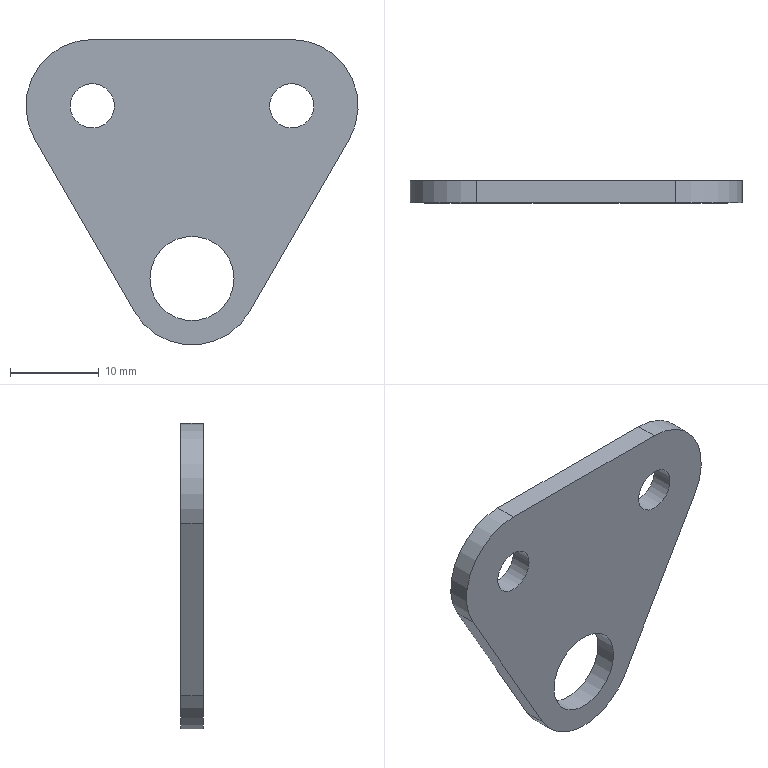Component | NX | 7 | 1 solid | 11 faces | box 37.5 x 2.5 x 34.49 mm | volume 1980 mm3 | cylinder 6 | plane 5 | commonest cylinder face diameters 15 x3 5 x2 9.5 x1
STEP:
#1=CARTESIAN_POINT('',(0.,0.,0.));
#2=DIRECTION('',(0.,0.,1.));
#3=DIRECTION('',(1.,0.,0.));
#4=AXIS2_PLACEMENT_3D('',#1,#2,#3);
#5=CARTESIAN_POINT('',(-395.181,171.749,-74.831));
#6=VERTEX_POINT('',#5);
#7=CARTESIAN_POINT('',(-388.686,171.749,-63.581));
#8=VERTEX_POINT('',#7);
#9=CARTESIAN_POINT('',(-388.686,171.749,-71.081));
#10=DIRECTION('',(0.,1.,0.));
#11=DIRECTION('',(-1.,0.,0.));
#12=AXIS2_PLACEMENT_3D('',#9,#10,#11);
#13=CIRCLE('',#12,7.5);
#14=CARTESIAN_POINT('',(-388.686,174.249,-71.081));
#15=DIRECTION('',(0.,-1.,0.));
#16=DIRECTION('',(-1.,0.,0.));
#17=AXIS2_PLACEMENT_3D('',#14,#15,#16);
#18=CYLINDRICAL_SURFACE('',#17,7.5);
#19=CARTESIAN_POINT('',(12.566,2.5));
#20=DIRECTION('',(-1.,0.));
#21=VECTOR('',#20,1.);
#22=LINE('',#19,#21);
#23=(GEOMETRIC_REPRESENTATION_CONTEXT(2)PARAMETRIC_REPRESENTATION_CONTEXT()REPRESENTATION_CONTEXT('',''));
#24=DEFINITIONAL_REPRESENTATION('',(#22),#23);
#25=PCURVE('',#18,#24);
#26=CARTESIAN_POINT('',(-388.686,171.749,-71.081));
#27=DIRECTION('',(0.,1.,0.));
#28=DIRECTION('',(1.,0.,0.));
#29=AXIS2_PLACEMENT_3D('',#26,#27,#28);
#30=PLANE('',#29);
#31=CARTESIAN_POINT('',(0.,0.));
#32=DIRECTION('',(-1.,0.));
#33=AXIS2_PLACEMENT_2D('',#31,#32);
#34=CIRCLE('',#33,7.5);
#35=(GEOMETRIC_REPRESENTATION_CONTEXT(2)PARAMETRIC_REPRESENTATION_CONTEXT()REPRESENTATION_CONTEXT('',''));
#36=DEFINITIONAL_REPRESENTATION('',(#34),#35);
#37=PCURVE('',#30,#36);
#38=SURFACE_CURVE('',#13,(#25,#37),.PCURVE_S1.);
#39=EDGE_CURVE('',#6,#8,#38,.T.);
#40=ORIENTED_EDGE('',*,*,#39,.T.);
#41=CARTESIAN_POINT('',(-388.686,174.249,-63.581));
#42=VERTEX_POINT('',#41);
#43=CARTESIAN_POINT('',(-388.686,174.249,-63.581));
#44=DIRECTION('',(0.,-1.,0.));
#45=VECTOR('',#44,1.);
#46=LINE('',#43,#45);
#47=CARTESIAN_POINT('',(4.712,0.));
#48=DIRECTION('',(0.,1.));
#49=VECTOR('',#48,1.);
#50=LINE('',#47,#49);
#51=(GEOMETRIC_REPRESENTATION_CONTEXT(2)PARAMETRIC_REPRESENTATION_CONTEXT()REPRESENTATION_CONTEXT('',''));
#52=DEFINITIONAL_REPRESENTATION('',(#50),#51);
#53=PCURVE('',#18,#52);
#54=CARTESIAN_POINT('',(-388.686,174.249,-63.581));
#55=DIRECTION('',(0.,0.,-1.));
#56=DIRECTION('',(0.,1.,0.));
#57=AXIS2_PLACEMENT_3D('',#54,#55,#56);
#58=PLANE('',#57);
#59=CARTESIAN_POINT('',(0.,0.));
#60=DIRECTION('',(-1.,0.));
#61=VECTOR('',#60,1.);
#62=LINE('',#59,#61);
#63=(GEOMETRIC_REPRESENTATION_CONTEXT(2)PARAMETRIC_REPRESENTATION_CONTEXT()REPRESENTATION_CONTEXT('',''));
#64=DEFINITIONAL_REPRESENTATION('',(#62),#63);
#65=PCURVE('',#58,#64);
#66=SURFACE_CURVE('',#46,(#53,#65),.PCURVE_S1.);
#67=EDGE_CURVE('',#42,#8,#66,.T.);
#68=ORIENTED_EDGE('',*,*,#67,.F.);
#69=CARTESIAN_POINT('',(-395.181,174.249,-74.831));
#70=VERTEX_POINT('',#69);
#71=CARTESIAN_POINT('',(-388.686,174.249,-71.081));
#72=DIRECTION('',(0.,1.,0.));
#73=DIRECTION('',(-1.,0.,0.));
#74=AXIS2_PLACEMENT_3D('',#71,#72,#73);
#75=CIRCLE('',#74,7.5);
#76=CARTESIAN_POINT('',(12.566,0.));
#77=DIRECTION('',(-1.,0.));
#78=VECTOR('',#77,1.);
#79=LINE('',#76,#78);
#80=(GEOMETRIC_REPRESENTATION_CONTEXT(2)PARAMETRIC_REPRESENTATION_CONTEXT()REPRESENTATION_CONTEXT('',''));
#81=DEFINITIONAL_REPRESENTATION('',(#79),#80);
#82=PCURVE('',#18,#81);
#83=CARTESIAN_POINT('',(-388.686,174.249,-71.081));
#84=DIRECTION('',(0.,1.,0.));
#85=DIRECTION('',(1.,0.,0.));
#86=AXIS2_PLACEMENT_3D('',#83,#84,#85);
#87=PLANE('',#86);
#88=CARTESIAN_POINT('',(0.,0.));
#89=DIRECTION('',(-1.,0.));
#90=AXIS2_PLACEMENT_2D('',#88,#89);
#91=CIRCLE('',#90,7.5);
#92=(GEOMETRIC_REPRESENTATION_CONTEXT(2)PARAMETRIC_REPRESENTATION_CONTEXT()REPRESENTATION_CONTEXT('',''));
#93=DEFINITIONAL_REPRESENTATION('',(#91),#92);
#94=PCURVE('',#87,#93);
#95=SURFACE_CURVE('',#75,(#82,#94),.PCURVE_S1.);
#96=EDGE_CURVE('',#70,#42,#95,.T.);
#97=ORIENTED_EDGE('',*,*,#96,.F.);
#98=CARTESIAN_POINT('',(-395.181,174.249,-74.831));
#99=DIRECTION('',(0.,-1.,0.));
#100=VECTOR('',#99,1.);
#101=LINE('',#98,#100);
#102=CARTESIAN_POINT('',(6.807,0.));
#103=DIRECTION('',(0.,1.));
#104=VECTOR('',#103,1.);
#105=LINE('',#102,#104);
#106=(GEOMETRIC_REPRESENTATION_CONTEXT(2)PARAMETRIC_REPRESENTATION_CONTEXT()REPRESENTATION_CONTEXT('',''));
#107=DEFINITIONAL_REPRESENTATION('',(#105),#106);
#108=PCURVE('',#18,#107);
#109=CARTESIAN_POINT('',(-383.931,174.249,-94.316));
#110=DIRECTION('',(0.866,0.,0.5));
#111=DIRECTION('',(0.5,0.,-0.866));
#112=AXIS2_PLACEMENT_3D('',#109,#110,#111);
#113=PLANE('',#112);
#114=CARTESIAN_POINT('',(-22.5,0.));
#115=DIRECTION('',(0.,-1.));
#116=VECTOR('',#115,1.);
#117=LINE('',#114,#116);
#118=(GEOMETRIC_REPRESENTATION_CONTEXT(2)PARAMETRIC_REPRESENTATION_CONTEXT()REPRESENTATION_CONTEXT('',''));
#119=DEFINITIONAL_REPRESENTATION('',(#117),#118);
#120=PCURVE('',#113,#119);
#121=SURFACE_CURVE('',#101,(#108,#120),.PCURVE_S1.);
#122=EDGE_CURVE('',#70,#6,#121,.T.);
#123=ORIENTED_EDGE('',*,*,#122,.T.);
#124=EDGE_LOOP('',(#40,#68,#97,#123));
#125=FACE_BOUND('',#124,.T.);
#126=ADVANCED_FACE('',(#125),#18,.T.);
#127=CARTESIAN_POINT('',(-366.186,171.749,-63.581));
#128=VERTEX_POINT('',#127);
#129=CARTESIAN_POINT('',(-388.686,171.749,-63.581));
#130=DIRECTION('',(1.,0.,0.));
#131=VECTOR('',#130,1.);
#132=LINE('',#129,#131);
#133=CARTESIAN_POINT('',(-2.5,0.));
#134=DIRECTION('',(0.,1.));
#135=VECTOR('',#134,1.);
#136=LINE('',#133,#135);
#137=(GEOMETRIC_REPRESENTATION_CONTEXT(2)PARAMETRIC_REPRESENTATION_CONTEXT()REPRESENTATION_CONTEXT('',''));
#138=DEFINITIONAL_REPRESENTATION('',(#136),#137);
#139=PCURVE('',#58,#138);
#140=CARTESIAN_POINT('',(0.,-7.5));
#141=DIRECTION('',(1.,0.));
#142=VECTOR('',#141,1.);
#143=LINE('',#140,#142);
#144=(GEOMETRIC_REPRESENTATION_CONTEXT(2)PARAMETRIC_REPRESENTATION_CONTEXT()REPRESENTATION_CONTEXT('',''));
#145=DEFINITIONAL_REPRESENTATION('',(#143),#144);
#146=PCURVE('',#30,#145);
#147=SURFACE_CURVE('',#132,(#139,#146),.PCURVE_S1.);
#148=EDGE_CURVE('',#8,#128,#147,.T.);
#149=ORIENTED_EDGE('',*,*,#148,.T.);
#150=CARTESIAN_POINT('',(-366.186,174.249,-63.581));
#151=VERTEX_POINT('',#150);
#152=CARTESIAN_POINT('',(-366.186,174.249,-63.581));
#153=DIRECTION('',(0.,-1.,0.));
#154=VECTOR('',#153,1.);
#155=LINE('',#152,#154);
#156=CARTESIAN_POINT('',(0.,22.5));
#157=DIRECTION('',(-1.,0.));
#158=VECTOR('',#157,1.);
#159=LINE('',#156,#158);
#160=(GEOMETRIC_REPRESENTATION_CONTEXT(2)PARAMETRIC_REPRESENTATION_CONTEXT()REPRESENTATION_CONTEXT('',''));
#161=DEFINITIONAL_REPRESENTATION('',(#159),#160);
#162=PCURVE('',#58,#161);
#163=CARTESIAN_POINT('',(-366.186,174.249,-71.081));
#164=DIRECTION('',(0.,-1.,0.));
#165=DIRECTION('',(-1.,0.,0.));
#166=AXIS2_PLACEMENT_3D('',#163,#164,#165);
#167=CYLINDRICAL_SURFACE('',#166,7.5);
#168=CARTESIAN_POINT('',(4.712,0.));
#169=DIRECTION('',(0.,1.));
#170=VECTOR('',#169,1.);
#171=LINE('',#168,#170);
#172=(GEOMETRIC_REPRESENTATION_CONTEXT(2)PARAMETRIC_REPRESENTATION_CONTEXT()REPRESENTATION_CONTEXT('',''));
#173=DEFINITIONAL_REPRESENTATION('',(#171),#172);
#174=PCURVE('',#167,#173);
#175=SURFACE_CURVE('',#155,(#162,#174),.PCURVE_S1.);
#176=EDGE_CURVE('',#151,#128,#175,.T.);
#177=ORIENTED_EDGE('',*,*,#176,.F.);
#178=CARTESIAN_POINT('',(-388.686,174.249,-63.581));
#179=DIRECTION('',(1.,0.,0.));
#180=VECTOR('',#179,1.);
#181=LINE('',#178,#180);
#182=CARTESIAN_POINT('',(0.,0.));
#183=DIRECTION('',(0.,1.));
#184=VECTOR('',#183,1.);
#185=LINE('',#182,#184);
#186=(GEOMETRIC_REPRESENTATION_CONTEXT(2)PARAMETRIC_REPRESENTATION_CONTEXT()REPRESENTATION_CONTEXT('',''));
#187=DEFINITIONAL_REPRESENTATION('',(#185),#186);
#188=PCURVE('',#58,#187);
#189=CARTESIAN_POINT('',(0.,-7.5));
#190=DIRECTION('',(1.,0.));
#191=VECTOR('',#190,1.);
#192=LINE('',#189,#191);
#193=(GEOMETRIC_REPRESENTATION_CONTEXT(2)PARAMETRIC_REPRESENTATION_CONTEXT()REPRESENTATION_CONTEXT('',''));
#194=DEFINITIONAL_REPRESENTATION('',(#192),#193);
#195=PCURVE('',#87,#194);
#196=SURFACE_CURVE('',#181,(#188,#195),.PCURVE_S1.);
#197=EDGE_CURVE('',#42,#151,#196,.T.);
#198=ORIENTED_EDGE('',*,*,#197,.F.);
#199=ORIENTED_EDGE('',*,*,#67,.T.);
#200=EDGE_LOOP('',(#149,#177,#198,#199));
#201=FACE_BOUND('',#200,.T.);
#202=ADVANCED_FACE('',(#201),#58,.F.);
#203=CARTESIAN_POINT('',(-359.69,171.749,-74.831));
#204=VERTEX_POINT('',#203);
#205=CARTESIAN_POINT('',(-366.186,171.749,-71.081));
#206=DIRECTION('',(0.,1.,0.));
#207=DIRECTION('',(-1.,0.,0.));
#208=AXIS2_PLACEMENT_3D('',#205,#206,#207);
#209=CIRCLE('',#208,7.5);
#210=CARTESIAN_POINT('',(6.283,2.5));
#211=DIRECTION('',(-1.,0.));
#212=VECTOR('',#211,1.);
#213=LINE('',#210,#212);
#214=(GEOMETRIC_REPRESENTATION_CONTEXT(2)PARAMETRIC_REPRESENTATION_CONTEXT()REPRESENTATION_CONTEXT('',''));
#215=DEFINITIONAL_REPRESENTATION('',(#213),#214);
#216=PCURVE('',#167,#215);
#217=CARTESIAN_POINT('',(22.5,0.));
#218=DIRECTION('',(-1.,0.));
#219=AXIS2_PLACEMENT_2D('',#217,#218);
#220=CIRCLE('',#219,7.5);
#221=(GEOMETRIC_REPRESENTATION_CONTEXT(2)PARAMETRIC_REPRESENTATION_CONTEXT()REPRESENTATION_CONTEXT('',''));
#222=DEFINITIONAL_REPRESENTATION('',(#220),#221);
#223=PCURVE('',#30,#222);
#224=SURFACE_CURVE('',#209,(#216,#223),.PCURVE_S1.);
#225=EDGE_CURVE('',#128,#204,#224,.T.);
#226=ORIENTED_EDGE('',*,*,#225,.T.);
#227=CARTESIAN_POINT('',(-359.69,174.249,-74.831));
#228=VERTEX_POINT('',#227);
#229=CARTESIAN_POINT('',(-359.69,174.249,-74.831));
#230=DIRECTION('',(0.,-1.,0.));
#231=VECTOR('',#230,1.);
#232=LINE('',#229,#231);
#233=CARTESIAN_POINT('',(2.618,0.));
#234=DIRECTION('',(0.,1.));
#235=VECTOR('',#234,1.);
#236=LINE('',#233,#235);
#237=(GEOMETRIC_REPRESENTATION_CONTEXT(2)PARAMETRIC_REPRESENTATION_CONTEXT()REPRESENTATION_CONTEXT('',''));
#238=DEFINITIONAL_REPRESENTATION('',(#236),#237);
#239=PCURVE('',#167,#238);
#240=CARTESIAN_POINT('',(-359.69,174.249,-74.831));
#241=DIRECTION('',(-0.866,0.,0.5));
#242=DIRECTION('',(0.5,0.,0.866));
#243=AXIS2_PLACEMENT_3D('',#240,#241,#242);
#244=PLANE('',#243);
#245=CARTESIAN_POINT('',(0.,0.));
#246=DIRECTION('',(0.,-1.));
#247=VECTOR('',#246,1.);
#248=LINE('',#245,#247);
#249=(GEOMETRIC_REPRESENTATION_CONTEXT(2)PARAMETRIC_REPRESENTATION_CONTEXT()REPRESENTATION_CONTEXT('',''));
#250=DEFINITIONAL_REPRESENTATION('',(#248),#249);
#251=PCURVE('',#244,#250);
#252=SURFACE_CURVE('',#232,(#239,#251),.PCURVE_S1.);
#253=EDGE_CURVE('',#228,#204,#252,.T.);
#254=ORIENTED_EDGE('',*,*,#253,.F.);
#255=CARTESIAN_POINT('',(-366.186,174.249,-71.081));
#256=DIRECTION('',(0.,1.,0.));
#257=DIRECTION('',(-1.,0.,0.));
#258=AXIS2_PLACEMENT_3D('',#255,#256,#257);
#259=CIRCLE('',#258,7.5);
#260=CARTESIAN_POINT('',(6.283,0.));
#261=DIRECTION('',(-1.,0.));
#262=VECTOR('',#261,1.);
#263=LINE('',#260,#262);
#264=(GEOMETRIC_REPRESENTATION_CONTEXT(2)PARAMETRIC_REPRESENTATION_CONTEXT()REPRESENTATION_CONTEXT('',''));
#265=DEFINITIONAL_REPRESENTATION('',(#263),#264);
#266=PCURVE('',#167,#265);
#267=CARTESIAN_POINT('',(22.5,0.));
#268=DIRECTION('',(-1.,0.));
#269=AXIS2_PLACEMENT_2D('',#267,#268);
#270=CIRCLE('',#269,7.5);
#271=(GEOMETRIC_REPRESENTATION_CONTEXT(2)PARAMETRIC_REPRESENTATION_CONTEXT()REPRESENTATION_CONTEXT('',''));
#272=DEFINITIONAL_REPRESENTATION('',(#270),#271);
#273=PCURVE('',#87,#272);
#274=SURFACE_CURVE('',#259,(#266,#273),.PCURVE_S1.);
#275=EDGE_CURVE('',#151,#228,#274,.T.);
#276=ORIENTED_EDGE('',*,*,#275,.F.);
#277=ORIENTED_EDGE('',*,*,#176,.T.);
#278=EDGE_LOOP('',(#226,#254,#276,#277));
#279=FACE_BOUND('',#278,.T.);
#280=ADVANCED_FACE('',(#279),#167,.T.);
#281=CARTESIAN_POINT('',(-370.94,171.749,-94.316));
#282=VERTEX_POINT('',#281);
#283=CARTESIAN_POINT('',(-359.69,171.749,-74.831));
#284=DIRECTION('',(-0.5,0.,-0.866));
#285=VECTOR('',#284,1.);
#286=LINE('',#283,#285);
#287=CARTESIAN_POINT('',(0.,-2.5));
#288=DIRECTION('',(-1.,0.));
#289=VECTOR('',#288,1.);
#290=LINE('',#287,#289);
#291=(GEOMETRIC_REPRESENTATION_CONTEXT(2)PARAMETRIC_REPRESENTATION_CONTEXT()REPRESENTATION_CONTEXT('',''));
#292=DEFINITIONAL_REPRESENTATION('',(#290),#291);
#293=PCURVE('',#244,#292);
#294=CARTESIAN_POINT('',(28.995,3.75));
#295=DIRECTION('',(-0.5,0.866));
#296=VECTOR('',#295,1.);
#297=LINE('',#294,#296);
#298=(GEOMETRIC_REPRESENTATION_CONTEXT(2)PARAMETRIC_REPRESENTATION_CONTEXT()REPRESENTATION_CONTEXT('',''));
#299=DEFINITIONAL_REPRESENTATION('',(#297),#298);
#300=PCURVE('',#30,#299);
#301=SURFACE_CURVE('',#286,(#293,#300),.PCURVE_S1.);
#302=EDGE_CURVE('',#204,#282,#301,.T.);
#303=ORIENTED_EDGE('',*,*,#302,.T.);
#304=CARTESIAN_POINT('',(-370.94,174.249,-94.316));
#305=VERTEX_POINT('',#304);
#306=CARTESIAN_POINT('',(-370.94,174.249,-94.316));
#307=DIRECTION('',(0.,-1.,0.));
#308=VECTOR('',#307,1.);
#309=LINE('',#306,#308);
#310=CARTESIAN_POINT('',(-22.5,0.));
#311=DIRECTION('',(0.,-1.));
#312=VECTOR('',#311,1.);
#313=LINE('',#310,#312);
#314=(GEOMETRIC_REPRESENTATION_CONTEXT(2)PARAMETRIC_REPRESENTATION_CONTEXT()REPRESENTATION_CONTEXT('',''));
#315=DEFINITIONAL_REPRESENTATION('',(#313),#314);
#316=PCURVE('',#244,#315);
#317=CARTESIAN_POINT('',(-377.436,174.249,-90.566));
#318=DIRECTION('',(0.,-1.,0.));
#319=DIRECTION('',(-1.,0.,0.));
#320=AXIS2_PLACEMENT_3D('',#317,#318,#319);
#321=CYLINDRICAL_SURFACE('',#320,7.5);
#322=CARTESIAN_POINT('',(2.618,0.));
#323=DIRECTION('',(0.,1.));
#324=VECTOR('',#323,1.);
#325=LINE('',#322,#324);
#326=(GEOMETRIC_REPRESENTATION_CONTEXT(2)PARAMETRIC_REPRESENTATION_CONTEXT()REPRESENTATION_CONTEXT('',''));
#327=DEFINITIONAL_REPRESENTATION('',(#325),#326);
#328=PCURVE('',#321,#327);
#329=SURFACE_CURVE('',#309,(#316,#328),.PCURVE_S1.);
#330=EDGE_CURVE('',#305,#282,#329,.T.);
#331=ORIENTED_EDGE('',*,*,#330,.F.);
#332=CARTESIAN_POINT('',(-359.69,174.249,-74.831));
#333=DIRECTION('',(-0.5,0.,-0.866));
#334=VECTOR('',#333,1.);
#335=LINE('',#332,#334);
#336=CARTESIAN_POINT('',(0.,0.));
#337=DIRECTION('',(-1.,0.));
#338=VECTOR('',#337,1.);
#339=LINE('',#336,#338);
#340=(GEOMETRIC_REPRESENTATION_CONTEXT(2)PARAMETRIC_REPRESENTATION_CONTEXT()REPRESENTATION_CONTEXT('',''));
#341=DEFINITIONAL_REPRESENTATION('',(#339),#340);
#342=PCURVE('',#244,#341);
#343=CARTESIAN_POINT('',(28.995,3.75));
#344=DIRECTION('',(-0.5,0.866));
#345=VECTOR('',#344,1.);
#346=LINE('',#343,#345);
#347=(GEOMETRIC_REPRESENTATION_CONTEXT(2)PARAMETRIC_REPRESENTATION_CONTEXT()REPRESENTATION_CONTEXT('',''));
#348=DEFINITIONAL_REPRESENTATION('',(#346),#347);
#349=PCURVE('',#87,#348);
#350=SURFACE_CURVE('',#335,(#342,#349),.PCURVE_S1.);
#351=EDGE_CURVE('',#228,#305,#350,.T.);
#352=ORIENTED_EDGE('',*,*,#351,.F.);
#353=ORIENTED_EDGE('',*,*,#253,.T.);
#354=EDGE_LOOP('',(#303,#331,#352,#353));
#355=FACE_BOUND('',#354,.T.);
#356=ADVANCED_FACE('',(#355),#244,.F.);
#357=CARTESIAN_POINT('',(-383.931,171.749,-94.316));
#358=VERTEX_POINT('',#357);
#359=CARTESIAN_POINT('',(-377.436,171.749,-90.566));
#360=DIRECTION('',(0.,1.,0.));
#361=DIRECTION('',(-1.,0.,0.));
#362=AXIS2_PLACEMENT_3D('',#359,#360,#361);
#363=CIRCLE('',#362,7.5);
#364=CARTESIAN_POINT('',(6.283,2.5));
#365=DIRECTION('',(-1.,0.));
#366=VECTOR('',#365,1.);
#367=LINE('',#364,#366);
#368=(GEOMETRIC_REPRESENTATION_CONTEXT(2)PARAMETRIC_REPRESENTATION_CONTEXT()REPRESENTATION_CONTEXT('',''));
#369=DEFINITIONAL_REPRESENTATION('',(#367),#368);
#370=PCURVE('',#321,#369);
#371=CARTESIAN_POINT('',(11.25,19.486));
#372=DIRECTION('',(-1.,0.));
#373=AXIS2_PLACEMENT_2D('',#371,#372);
#374=CIRCLE('',#373,7.5);
#375=(GEOMETRIC_REPRESENTATION_CONTEXT(2)PARAMETRIC_REPRESENTATION_CONTEXT()REPRESENTATION_CONTEXT('',''));
#376=DEFINITIONAL_REPRESENTATION('',(#374),#375);
#377=PCURVE('',#30,#376);
#378=SURFACE_CURVE('',#363,(#370,#377),.PCURVE_S1.);
#379=EDGE_CURVE('',#282,#358,#378,.T.);
#380=ORIENTED_EDGE('',*,*,#379,.T.);
#381=CARTESIAN_POINT('',(-383.931,174.249,-94.316));
#382=VERTEX_POINT('',#381);
#383=CARTESIAN_POINT('',(-383.931,174.249,-94.316));
#384=DIRECTION('',(0.,-1.,0.));
#385=VECTOR('',#384,1.);
#386=LINE('',#383,#385);
#387=CARTESIAN_POINT('',(0.5236,0.));
#388=DIRECTION('',(0.,1.));
#389=VECTOR('',#388,1.);
#390=LINE('',#387,#389);
#391=(GEOMETRIC_REPRESENTATION_CONTEXT(2)PARAMETRIC_REPRESENTATION_CONTEXT()REPRESENTATION_CONTEXT('',''));
#392=DEFINITIONAL_REPRESENTATION('',(#390),#391);
#393=PCURVE('',#321,#392);
#394=CARTESIAN_POINT('',(0.,0.));
#395=DIRECTION('',(0.,-1.));
#396=VECTOR('',#395,1.);
#397=LINE('',#394,#396);
#398=(GEOMETRIC_REPRESENTATION_CONTEXT(2)PARAMETRIC_REPRESENTATION_CONTEXT()REPRESENTATION_CONTEXT('',''));
#399=DEFINITIONAL_REPRESENTATION('',(#397),#398);
#400=PCURVE('',#113,#399);
#401=SURFACE_CURVE('',#386,(#393,#400),.PCURVE_S1.);
#402=EDGE_CURVE('',#382,#358,#401,.T.);
#403=ORIENTED_EDGE('',*,*,#402,.F.);
#404=CARTESIAN_POINT('',(-377.436,174.249,-90.566));
#405=DIRECTION('',(0.,1.,0.));
#406=DIRECTION('',(-1.,0.,0.));
#407=AXIS2_PLACEMENT_3D('',#404,#405,#406);
#408=CIRCLE('',#407,7.5);
#409=CARTESIAN_POINT('',(6.283,0.));
#410=DIRECTION('',(-1.,0.));
#411=VECTOR('',#410,1.);
#412=LINE('',#409,#411);
#413=(GEOMETRIC_REPRESENTATION_CONTEXT(2)PARAMETRIC_REPRESENTATION_CONTEXT()REPRESENTATION_CONTEXT('',''));
#414=DEFINITIONAL_REPRESENTATION('',(#412),#413);
#415=PCURVE('',#321,#414);
#416=CARTESIAN_POINT('',(11.25,19.486));
#417=DIRECTION('',(-1.,0.));
#418=AXIS2_PLACEMENT_2D('',#416,#417);
#419=CIRCLE('',#418,7.5);
#420=(GEOMETRIC_REPRESENTATION_CONTEXT(2)PARAMETRIC_REPRESENTATION_CONTEXT()REPRESENTATION_CONTEXT('',''));
#421=DEFINITIONAL_REPRESENTATION('',(#419),#420);
#422=PCURVE('',#87,#421);
#423=SURFACE_CURVE('',#408,(#415,#422),.PCURVE_S1.);
#424=EDGE_CURVE('',#305,#382,#423,.T.);
#425=ORIENTED_EDGE('',*,*,#424,.F.);
#426=ORIENTED_EDGE('',*,*,#330,.T.);
#427=EDGE_LOOP('',(#380,#403,#425,#426));
#428=FACE_BOUND('',#427,.T.);
#429=ADVANCED_FACE('',(#428),#321,.T.);
#430=CARTESIAN_POINT('',(-391.186,174.249,-71.081));
#431=VERTEX_POINT('',#430);
#432=CARTESIAN_POINT('',(-388.686,174.249,-71.081));
#433=DIRECTION('',(0.,-1.,0.));
#434=DIRECTION('',(-1.,0.,0.));
#435=AXIS2_PLACEMENT_3D('',#432,#433,#434);
#436=CIRCLE('',#435,2.5);
#437=CARTESIAN_POINT('',(-388.686,174.249,-71.081));
#438=DIRECTION('',(0.,-1.,0.));
#439=DIRECTION('',(-1.,0.,0.));
#440=AXIS2_PLACEMENT_3D('',#437,#438,#439);
#441=CYLINDRICAL_SURFACE('',#440,2.5);
#442=CARTESIAN_POINT('',(0.,0.));
#443=DIRECTION('',(1.,0.));
#444=VECTOR('',#443,1.);
#445=LINE('',#442,#444);
#446=(GEOMETRIC_REPRESENTATION_CONTEXT(2)PARAMETRIC_REPRESENTATION_CONTEXT()REPRESENTATION_CONTEXT('',''));
#447=DEFINITIONAL_REPRESENTATION('',(#445),#446);
#448=PCURVE('',#441,#447);
#449=CARTESIAN_POINT('',(-2.5,0.));
#450=CARTESIAN_POINT('',(-2.5,4.33));
#451=CARTESIAN_POINT('',(1.25,2.165));
#452=CARTESIAN_POINT('',(5.,0.));
#453=CARTESIAN_POINT('',(1.25,-2.165));
#454=CARTESIAN_POINT('',(-2.5,-4.33));
#455=CARTESIAN_POINT('',(-2.5,0.));
#456=(BOUNDED_CURVE()B_SPLINE_CURVE(2,(#449,#450,#451,#452,#453,#454,#455),.UNSPECIFIED.,.T.,.F.)B_SPLINE_CURVE_WITH_KNOTS((1,2,2,2,2,1),(-2.094,0.,2.094,4.189,6.283,8.378),.UNSPECIFIED.)CURVE()GEOMETRIC_REPRESENTATION_ITEM()RATIONAL_B_SPLINE_CURVE((1.,0.5,1.,0.5,1.,0.5,1.))REPRESENTATION_ITEM(''));
#457=(GEOMETRIC_REPRESENTATION_CONTEXT(2)PARAMETRIC_REPRESENTATION_CONTEXT()REPRESENTATION_CONTEXT('',''));
#458=DEFINITIONAL_REPRESENTATION('',(#456),#457);
#459=PCURVE('',#87,#458);
#460=SURFACE_CURVE('',#436,(#448,#459),.PCURVE_S1.);
#461=EDGE_CURVE('',#431,#431,#460,.T.);
#462=ORIENTED_EDGE('',*,*,#461,.T.);
#463=CARTESIAN_POINT('',(-391.186,171.749,-71.081));
#464=VERTEX_POINT('',#463);
#465=CARTESIAN_POINT('',(-391.186,174.249,-71.081));
#466=CARTESIAN_POINT('',(-391.186,171.749,-71.081));
#467=B_SPLINE_CURVE_WITH_KNOTS('',1,(#465,#466),.UNSPECIFIED.,.F.,.F.,(2,2),(0.,2.5),.PIECEWISE_BEZIER_KNOTS.);
#468=CARTESIAN_POINT('',(6.283,0.));
#469=DIRECTION('',(0.,1.));
#470=VECTOR('',#469,1.);
#471=LINE('',#468,#470);
#472=(GEOMETRIC_REPRESENTATION_CONTEXT(2)PARAMETRIC_REPRESENTATION_CONTEXT()REPRESENTATION_CONTEXT('',''));
#473=DEFINITIONAL_REPRESENTATION('',(#471),#472);
#474=PCURVE('',#441,#473);
#475=CARTESIAN_POINT('',(0.,0.));
#476=DIRECTION('',(0.,1.));
#477=VECTOR('',#476,1.);
#478=LINE('',#475,#477);
#479=(GEOMETRIC_REPRESENTATION_CONTEXT(2)PARAMETRIC_REPRESENTATION_CONTEXT()REPRESENTATION_CONTEXT('',''));
#480=DEFINITIONAL_REPRESENTATION('',(#478),#479);
#481=PCURVE('',#441,#480);
#482=SEAM_CURVE('',#467,(#474,#481),.PCURVE_S1.);
#483=EDGE_CURVE('',#431,#464,#482,.T.);
#484=ORIENTED_EDGE('',*,*,#483,.T.);
#485=CARTESIAN_POINT('',(-388.686,171.749,-71.081));
#486=DIRECTION('',(0.,-1.,0.));
#487=DIRECTION('',(-1.,0.,0.));
#488=AXIS2_PLACEMENT_3D('',#485,#486,#487);
#489=CIRCLE('',#488,2.5);
#490=CARTESIAN_POINT('',(0.,2.5));
#491=DIRECTION('',(1.,0.));
#492=VECTOR('',#491,1.);
#493=LINE('',#490,#492);
#494=(GEOMETRIC_REPRESENTATION_CONTEXT(2)PARAMETRIC_REPRESENTATION_CONTEXT()REPRESENTATION_CONTEXT('',''));
#495=DEFINITIONAL_REPRESENTATION('',(#493),#494);
#496=PCURVE('',#441,#495);
#497=CARTESIAN_POINT('',(-2.5,0.));
#498=CARTESIAN_POINT('',(-2.5,4.33));
#499=CARTESIAN_POINT('',(1.25,2.165));
#500=CARTESIAN_POINT('',(5.,0.));
#501=CARTESIAN_POINT('',(1.25,-2.165));
#502=CARTESIAN_POINT('',(-2.5,-4.33));
#503=CARTESIAN_POINT('',(-2.5,0.));
#504=(BOUNDED_CURVE()B_SPLINE_CURVE(2,(#497,#498,#499,#500,#501,#502,#503),.UNSPECIFIED.,.T.,.F.)B_SPLINE_CURVE_WITH_KNOTS((1,2,2,2,2,1),(-2.094,0.,2.094,4.189,6.283,8.378),.UNSPECIFIED.)CURVE()GEOMETRIC_REPRESENTATION_ITEM()RATIONAL_B_SPLINE_CURVE((1.,0.5,1.,0.5,1.,0.5,1.))REPRESENTATION_ITEM(''));
#505=(GEOMETRIC_REPRESENTATION_CONTEXT(2)PARAMETRIC_REPRESENTATION_CONTEXT()REPRESENTATION_CONTEXT('',''));
#506=DEFINITIONAL_REPRESENTATION('',(#504),#505);
#507=PCURVE('',#30,#506);
#508=SURFACE_CURVE('',#489,(#496,#507),.PCURVE_S1.);
#509=EDGE_CURVE('',#464,#464,#508,.T.);
#510=ORIENTED_EDGE('',*,*,#509,.F.);
#511=ORIENTED_EDGE('',*,*,#483,.F.);
#512=EDGE_LOOP('',(#462,#484,#510,#511));
#513=FACE_BOUND('',#512,.F.);
#514=ADVANCED_FACE('',(#513),#441,.F.);
#515=CARTESIAN_POINT('',(-368.686,174.249,-71.081));
#516=VERTEX_POINT('',#515);
#517=CARTESIAN_POINT('',(-366.186,174.249,-71.081));
#518=DIRECTION('',(0.,-1.,0.));
#519=DIRECTION('',(-1.,0.,0.));
#520=AXIS2_PLACEMENT_3D('',#517,#518,#519);
#521=CIRCLE('',#520,2.5);
#522=CARTESIAN_POINT('',(-366.186,174.249,-71.081));
#523=DIRECTION('',(0.,-1.,0.));
#524=DIRECTION('',(-1.,0.,0.));
#525=AXIS2_PLACEMENT_3D('',#522,#523,#524);
#526=CYLINDRICAL_SURFACE('',#525,2.5);
#527=CARTESIAN_POINT('',(0.,0.));
#528=DIRECTION('',(1.,0.));
#529=VECTOR('',#528,1.);
#530=LINE('',#527,#529);
#531=(GEOMETRIC_REPRESENTATION_CONTEXT(2)PARAMETRIC_REPRESENTATION_CONTEXT()REPRESENTATION_CONTEXT('',''));
#532=DEFINITIONAL_REPRESENTATION('',(#530),#531);
#533=PCURVE('',#526,#532);
#534=CARTESIAN_POINT('',(20.,0.));
#535=CARTESIAN_POINT('',(20.,4.33));
#536=CARTESIAN_POINT('',(23.75,2.165));
#537=CARTESIAN_POINT('',(27.5,0.));
#538=CARTESIAN_POINT('',(23.75,-2.165));
#539=CARTESIAN_POINT('',(20.,-4.33));
#540=CARTESIAN_POINT('',(20.,0.));
#541=(BOUNDED_CURVE()B_SPLINE_CURVE(2,(#534,#535,#536,#537,#538,#539,#540),.UNSPECIFIED.,.T.,.F.)B_SPLINE_CURVE_WITH_KNOTS((1,2,2,2,2,1),(-2.094,0.,2.094,4.189,6.283,8.378),.UNSPECIFIED.)CURVE()GEOMETRIC_REPRESENTATION_ITEM()RATIONAL_B_SPLINE_CURVE((1.,0.5,1.,0.5,1.,0.5,1.))REPRESENTATION_ITEM(''));
#542=(GEOMETRIC_REPRESENTATION_CONTEXT(2)PARAMETRIC_REPRESENTATION_CONTEXT()REPRESENTATION_CONTEXT('',''));
#543=DEFINITIONAL_REPRESENTATION('',(#541),#542);
#544=PCURVE('',#87,#543);
#545=SURFACE_CURVE('',#521,(#533,#544),.PCURVE_S1.);
#546=EDGE_CURVE('',#516,#516,#545,.T.);
#547=ORIENTED_EDGE('',*,*,#546,.T.);
#548=CARTESIAN_POINT('',(-368.686,171.749,-71.081));
#549=VERTEX_POINT('',#548);
#550=CARTESIAN_POINT('',(-368.686,174.249,-71.081));
#551=CARTESIAN_POINT('',(-368.686,171.749,-71.081));
#552=B_SPLINE_CURVE_WITH_KNOTS('',1,(#550,#551),.UNSPECIFIED.,.F.,.F.,(2,2),(0.,2.5),.PIECEWISE_BEZIER_KNOTS.);
#553=CARTESIAN_POINT('',(6.283,0.));
#554=DIRECTION('',(0.,1.));
#555=VECTOR('',#554,1.);
#556=LINE('',#553,#555);
#557=(GEOMETRIC_REPRESENTATION_CONTEXT(2)PARAMETRIC_REPRESENTATION_CONTEXT()REPRESENTATION_CONTEXT('',''));
#558=DEFINITIONAL_REPRESENTATION('',(#556),#557);
#559=PCURVE('',#526,#558);
#560=CARTESIAN_POINT('',(0.,0.));
#561=DIRECTION('',(0.,1.));
#562=VECTOR('',#561,1.);
#563=LINE('',#560,#562);
#564=(GEOMETRIC_REPRESENTATION_CONTEXT(2)PARAMETRIC_REPRESENTATION_CONTEXT()REPRESENTATION_CONTEXT('',''));
#565=DEFINITIONAL_REPRESENTATION('',(#563),#564);
#566=PCURVE('',#526,#565);
#567=SEAM_CURVE('',#552,(#559,#566),.PCURVE_S1.);
#568=EDGE_CURVE('',#516,#549,#567,.T.);
#569=ORIENTED_EDGE('',*,*,#568,.T.);
#570=CARTESIAN_POINT('',(-366.186,171.749,-71.081));
#571=DIRECTION('',(0.,-1.,0.));
#572=DIRECTION('',(-1.,0.,0.));
#573=AXIS2_PLACEMENT_3D('',#570,#571,#572);
#574=CIRCLE('',#573,2.5);
#575=CARTESIAN_POINT('',(0.,2.5));
#576=DIRECTION('',(1.,0.));
#577=VECTOR('',#576,1.);
#578=LINE('',#575,#577);
#579=(GEOMETRIC_REPRESENTATION_CONTEXT(2)PARAMETRIC_REPRESENTATION_CONTEXT()REPRESENTATION_CONTEXT('',''));
#580=DEFINITIONAL_REPRESENTATION('',(#578),#579);
#581=PCURVE('',#526,#580);
#582=CARTESIAN_POINT('',(20.,0.));
#583=CARTESIAN_POINT('',(20.,4.33));
#584=CARTESIAN_POINT('',(23.75,2.165));
#585=CARTESIAN_POINT('',(27.5,0.));
#586=CARTESIAN_POINT('',(23.75,-2.165));
#587=CARTESIAN_POINT('',(20.,-4.33));
#588=CARTESIAN_POINT('',(20.,0.));
#589=(BOUNDED_CURVE()B_SPLINE_CURVE(2,(#582,#583,#584,#585,#586,#587,#588),.UNSPECIFIED.,.T.,.F.)B_SPLINE_CURVE_WITH_KNOTS((1,2,2,2,2,1),(-2.094,0.,2.094,4.189,6.283,8.378),.UNSPECIFIED.)CURVE()GEOMETRIC_REPRESENTATION_ITEM()RATIONAL_B_SPLINE_CURVE((1.,0.5,1.,0.5,1.,0.5,1.))REPRESENTATION_ITEM(''));
#590=(GEOMETRIC_REPRESENTATION_CONTEXT(2)PARAMETRIC_REPRESENTATION_CONTEXT()REPRESENTATION_CONTEXT('',''));
#591=DEFINITIONAL_REPRESENTATION('',(#589),#590);
#592=PCURVE('',#30,#591);
#593=SURFACE_CURVE('',#574,(#581,#592),.PCURVE_S1.);
#594=EDGE_CURVE('',#549,#549,#593,.T.);
#595=ORIENTED_EDGE('',*,*,#594,.F.);
#596=ORIENTED_EDGE('',*,*,#568,.F.);
#597=EDGE_LOOP('',(#547,#569,#595,#596));
#598=FACE_BOUND('',#597,.F.);
#599=ADVANCED_FACE('',(#598),#526,.F.);
#600=CARTESIAN_POINT('',(-383.931,171.749,-94.316));
#601=DIRECTION('',(-0.5,0.,0.866));
#602=VECTOR('',#601,1.);
#603=LINE('',#600,#602);
#604=CARTESIAN_POINT('',(0.,-2.5));
#605=DIRECTION('',(-1.,0.));
#606=VECTOR('',#605,1.);
#607=LINE('',#604,#606);
#608=(GEOMETRIC_REPRESENTATION_CONTEXT(2)PARAMETRIC_REPRESENTATION_CONTEXT()REPRESENTATION_CONTEXT('',''));
#609=DEFINITIONAL_REPRESENTATION('',(#607),#608);
#610=PCURVE('',#113,#609);
#611=CARTESIAN_POINT('',(4.755,23.236));
#612=DIRECTION('',(-0.5,-0.866));
#613=VECTOR('',#612,1.);
#614=LINE('',#611,#613);
#615=(GEOMETRIC_REPRESENTATION_CONTEXT(2)PARAMETRIC_REPRESENTATION_CONTEXT()REPRESENTATION_CONTEXT('',''));
#616=DEFINITIONAL_REPRESENTATION('',(#614),#615);
#617=PCURVE('',#30,#616);
#618=SURFACE_CURVE('',#603,(#610,#617),.PCURVE_S1.);
#619=EDGE_CURVE('',#358,#6,#618,.T.);
#620=ORIENTED_EDGE('',*,*,#619,.T.);
#621=ORIENTED_EDGE('',*,*,#122,.F.);
#622=CARTESIAN_POINT('',(-383.931,174.249,-94.316));
#623=DIRECTION('',(-0.5,0.,0.866));
#624=VECTOR('',#623,1.);
#625=LINE('',#622,#624);
#626=CARTESIAN_POINT('',(0.,0.));
#627=DIRECTION('',(-1.,0.));
#628=VECTOR('',#627,1.);
#629=LINE('',#626,#628);
#630=(GEOMETRIC_REPRESENTATION_CONTEXT(2)PARAMETRIC_REPRESENTATION_CONTEXT()REPRESENTATION_CONTEXT('',''));
#631=DEFINITIONAL_REPRESENTATION('',(#629),#630);
#632=PCURVE('',#113,#631);
#633=CARTESIAN_POINT('',(4.755,23.236));
#634=DIRECTION('',(-0.5,-0.866));
#635=VECTOR('',#634,1.);
#636=LINE('',#633,#635);
#637=(GEOMETRIC_REPRESENTATION_CONTEXT(2)PARAMETRIC_REPRESENTATION_CONTEXT()REPRESENTATION_CONTEXT('',''));
#638=DEFINITIONAL_REPRESENTATION('',(#636),#637);
#639=PCURVE('',#87,#638);
#640=SURFACE_CURVE('',#625,(#632,#639),.PCURVE_S1.);
#641=EDGE_CURVE('',#382,#70,#640,.T.);
#642=ORIENTED_EDGE('',*,*,#641,.F.);
#643=ORIENTED_EDGE('',*,*,#402,.T.);
#644=EDGE_LOOP('',(#620,#621,#642,#643));
#645=FACE_BOUND('',#644,.T.);
#646=ADVANCED_FACE('',(#645),#113,.F.);
#647=CARTESIAN_POINT('',(-382.186,174.249,-90.566));
#648=VERTEX_POINT('',#647);
#649=CARTESIAN_POINT('',(-377.436,174.249,-90.566));
#650=DIRECTION('',(0.,-1.,0.));
#651=DIRECTION('',(-1.,0.,0.));
#652=AXIS2_PLACEMENT_3D('',#649,#650,#651);
#653=CIRCLE('',#652,4.75);
#654=CARTESIAN_POINT('',(-377.436,174.249,-90.566));
#655=DIRECTION('',(0.,-1.,0.));
#656=DIRECTION('',(-1.,0.,0.));
#657=AXIS2_PLACEMENT_3D('',#654,#655,#656);
#658=CYLINDRICAL_SURFACE('',#657,4.75);
#659=CARTESIAN_POINT('',(0.,0.));
#660=DIRECTION('',(1.,0.));
#661=VECTOR('',#660,1.);
#662=LINE('',#659,#661);
#663=(GEOMETRIC_REPRESENTATION_CONTEXT(2)PARAMETRIC_REPRESENTATION_CONTEXT()REPRESENTATION_CONTEXT('',''));
#664=DEFINITIONAL_REPRESENTATION('',(#662),#663);
#665=PCURVE('',#658,#664);
#666=CARTESIAN_POINT('',(6.5,19.486));
#667=CARTESIAN_POINT('',(6.5,27.713));
#668=CARTESIAN_POINT('',(13.625,23.599));
#669=CARTESIAN_POINT('',(20.75,19.486));
#670=CARTESIAN_POINT('',(13.625,15.372));
#671=CARTESIAN_POINT('',(6.5,11.258));
#672=CARTESIAN_POINT('',(6.5,19.486));
#673=(BOUNDED_CURVE()B_SPLINE_CURVE(2,(#666,#667,#668,#669,#670,#671,#672),.UNSPECIFIED.,.T.,.F.)B_SPLINE_CURVE_WITH_KNOTS((1,2,2,2,2,1),(-2.094,0.,2.094,4.189,6.283,8.378),.UNSPECIFIED.)CURVE()GEOMETRIC_REPRESENTATION_ITEM()RATIONAL_B_SPLINE_CURVE((1.,0.5,1.,0.5,1.,0.5,1.))REPRESENTATION_ITEM(''));
#674=(GEOMETRIC_REPRESENTATION_CONTEXT(2)PARAMETRIC_REPRESENTATION_CONTEXT()REPRESENTATION_CONTEXT('',''));
#675=DEFINITIONAL_REPRESENTATION('',(#673),#674);
#676=PCURVE('',#87,#675);
#677=SURFACE_CURVE('',#653,(#665,#676),.PCURVE_S1.);
#678=EDGE_CURVE('',#648,#648,#677,.T.);
#679=ORIENTED_EDGE('',*,*,#678,.T.);
#680=CARTESIAN_POINT('',(-382.186,171.749,-90.566));
#681=VERTEX_POINT('',#680);
#682=CARTESIAN_POINT('',(-382.186,174.249,-90.566));
#683=CARTESIAN_POINT('',(-382.186,171.749,-90.566));
#684=B_SPLINE_CURVE_WITH_KNOTS('',1,(#682,#683),.UNSPECIFIED.,.F.,.F.,(2,2),(0.,2.5),.PIECEWISE_BEZIER_KNOTS.);
#685=CARTESIAN_POINT('',(6.283,0.));
#686=DIRECTION('',(0.,1.));
#687=VECTOR('',#686,1.);
#688=LINE('',#685,#687);
#689=(GEOMETRIC_REPRESENTATION_CONTEXT(2)PARAMETRIC_REPRESENTATION_CONTEXT()REPRESENTATION_CONTEXT('',''));
#690=DEFINITIONAL_REPRESENTATION('',(#688),#689);
#691=PCURVE('',#658,#690);
#692=CARTESIAN_POINT('',(0.,0.));
#693=DIRECTION('',(0.,1.));
#694=VECTOR('',#693,1.);
#695=LINE('',#692,#694);
#696=(GEOMETRIC_REPRESENTATION_CONTEXT(2)PARAMETRIC_REPRESENTATION_CONTEXT()REPRESENTATION_CONTEXT('',''));
#697=DEFINITIONAL_REPRESENTATION('',(#695),#696);
#698=PCURVE('',#658,#697);
#699=SEAM_CURVE('',#684,(#691,#698),.PCURVE_S1.);
#700=EDGE_CURVE('',#648,#681,#699,.T.);
#701=ORIENTED_EDGE('',*,*,#700,.T.);
#702=CARTESIAN_POINT('',(-377.436,171.749,-90.566));
#703=DIRECTION('',(0.,-1.,0.));
#704=DIRECTION('',(-1.,0.,0.));
#705=AXIS2_PLACEMENT_3D('',#702,#703,#704);
#706=CIRCLE('',#705,4.75);
#707=CARTESIAN_POINT('',(0.,2.5));
#708=DIRECTION('',(1.,0.));
#709=VECTOR('',#708,1.);
#710=LINE('',#707,#709);
#711=(GEOMETRIC_REPRESENTATION_CONTEXT(2)PARAMETRIC_REPRESENTATION_CONTEXT()REPRESENTATION_CONTEXT('',''));
#712=DEFINITIONAL_REPRESENTATION('',(#710),#711);
#713=PCURVE('',#658,#712);
#714=CARTESIAN_POINT('',(6.5,19.486));
#715=CARTESIAN_POINT('',(6.5,27.713));
#716=CARTESIAN_POINT('',(13.625,23.599));
#717=CARTESIAN_POINT('',(20.75,19.486));
#718=CARTESIAN_POINT('',(13.625,15.372));
#719=CARTESIAN_POINT('',(6.5,11.258));
#720=CARTESIAN_POINT('',(6.5,19.486));
#721=(BOUNDED_CURVE()B_SPLINE_CURVE(2,(#714,#715,#716,#717,#718,#719,#720),.UNSPECIFIED.,.T.,.F.)B_SPLINE_CURVE_WITH_KNOTS((1,2,2,2,2,1),(-2.094,0.,2.094,4.189,6.283,8.378),.UNSPECIFIED.)CURVE()GEOMETRIC_REPRESENTATION_ITEM()RATIONAL_B_SPLINE_CURVE((1.,0.5,1.,0.5,1.,0.5,1.))REPRESENTATION_ITEM(''));
#722=(GEOMETRIC_REPRESENTATION_CONTEXT(2)PARAMETRIC_REPRESENTATION_CONTEXT()REPRESENTATION_CONTEXT('',''));
#723=DEFINITIONAL_REPRESENTATION('',(#721),#722);
#724=PCURVE('',#30,#723);
#725=SURFACE_CURVE('',#706,(#713,#724),.PCURVE_S1.);
#726=EDGE_CURVE('',#681,#681,#725,.T.);
#727=ORIENTED_EDGE('',*,*,#726,.F.);
#728=ORIENTED_EDGE('',*,*,#700,.F.);
#729=EDGE_LOOP('',(#679,#701,#727,#728));
#730=FACE_BOUND('',#729,.F.);
#731=ADVANCED_FACE('',(#730),#658,.F.);
#732=ORIENTED_EDGE('',*,*,#96,.T.);
#733=ORIENTED_EDGE('',*,*,#197,.T.);
#734=ORIENTED_EDGE('',*,*,#275,.T.);
#735=ORIENTED_EDGE('',*,*,#351,.T.);
#736=ORIENTED_EDGE('',*,*,#424,.T.);
#737=ORIENTED_EDGE('',*,*,#641,.T.);
#738=EDGE_LOOP('',(#732,#733,#734,#735,#736,#737));
#739=FACE_BOUND('',#738,.T.);
#740=ORIENTED_EDGE('',*,*,#546,.T.);
#741=EDGE_LOOP('',(#740));
#742=FACE_BOUND('',#741,.T.);
#743=ORIENTED_EDGE('',*,*,#461,.T.);
#744=EDGE_LOOP('',(#743));
#745=FACE_BOUND('',#744,.T.);
#746=ORIENTED_EDGE('',*,*,#678,.T.);
#747=EDGE_LOOP('',(#746));
#748=FACE_BOUND('',#747,.T.);
#749=ADVANCED_FACE('',(#739,#742,#745,#748),#87,.T.);
#750=ORIENTED_EDGE('',*,*,#39,.F.);
#751=ORIENTED_EDGE('',*,*,#619,.F.);
#752=ORIENTED_EDGE('',*,*,#379,.F.);
#753=ORIENTED_EDGE('',*,*,#302,.F.);
#754=ORIENTED_EDGE('',*,*,#225,.F.);
#755=ORIENTED_EDGE('',*,*,#148,.F.);
#756=EDGE_LOOP('',(#750,#751,#752,#753,#754,#755));
#757=FACE_BOUND('',#756,.T.);
#758=ORIENTED_EDGE('',*,*,#594,.F.);
#759=EDGE_LOOP('',(#758));
#760=FACE_BOUND('',#759,.T.);
#761=ORIENTED_EDGE('',*,*,#509,.F.);
#762=EDGE_LOOP('',(#761));
#763=FACE_BOUND('',#762,.T.);
#764=ORIENTED_EDGE('',*,*,#726,.F.);
#765=EDGE_LOOP('',(#764));
#766=FACE_BOUND('',#765,.T.);
#767=ADVANCED_FACE('',(#757,#760,#763,#766),#30,.F.);
#768=CLOSED_SHELL('',(#126,#202,#280,#356,#429,#514,#599,#646,#731,#749,#767));
#769=MANIFOLD_SOLID_BREP('',#768);
#770=(LENGTH_UNIT()NAMED_UNIT(*)SI_UNIT(.MILLI.,.METRE.));
#771=UNCERTAINTY_MEASURE_WITH_UNIT(LENGTH_MEASURE(0.000002),#770,'','');
#772=(NAMED_UNIT(*)PLANE_ANGLE_UNIT()SI_UNIT($,.RADIAN.));
#773=(NAMED_UNIT(*)SI_UNIT($,.STERADIAN.)SOLID_ANGLE_UNIT());
#774=(GEOMETRIC_REPRESENTATION_CONTEXT(3)GLOBAL_UNCERTAINTY_ASSIGNED_CONTEXT((#771))GLOBAL_UNIT_ASSIGNED_CONTEXT((#770,#772,#773))REPRESENTATION_CONTEXT('',''));
#775=ADVANCED_BREP_SHAPE_REPRESENTATION('',(#4,#769),#774);